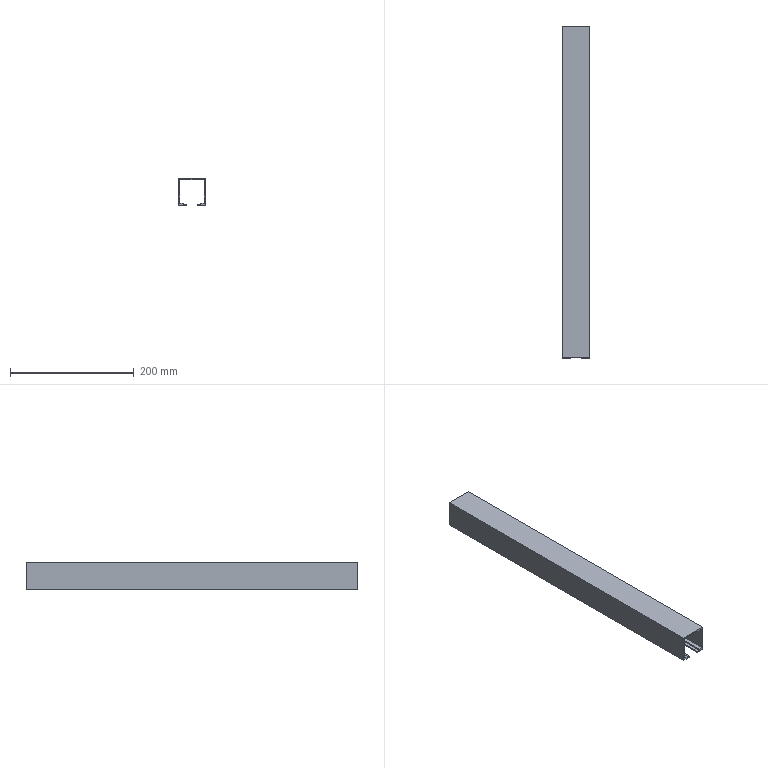Component | SolidWorks | SquareAluminumTube-2 | 1 solid | 18 faces | box 44 x 536 x 44 mm | volume 173664 mm3 | plane 18
build123d program:
from build123d import *

# Parameters (mm, degrees)
BOSS_EXTRUDE1_DEPTH = 536


with BuildPart() as part:
    # Sketch1 → Boss-Extrude1 (new body)
    with BuildSketch(Plane.XY):
        Polygon((-20, -18), (-20, 20), (20, 20), (20, -18), (14, -18), (14, -20), (9, -20), (9, -22), (22, -22), (22, 22), (-22, 22), (-22, -22), (-9, -22), (-9, -20), (-14, -20), (-14, -18), align=None)
    extrude(amount=BOSS_EXTRUDE1_DEPTH)


solid = part.part

# Placed as in the assembly
solid = solid.moved(Location((-67.793, 523.197, 1764.064), (90, 0, 0)))
STEP:
#1=CARTESIAN_POINT('',(-3.535,-0.5041,68.585));
#2=VERTEX_POINT('',#1);
#3=CARTESIAN_POINT('',(-3.535,-0.5041,70.317));
#4=VERTEX_POINT('',#3);
#5=CARTESIAN_POINT('',(-3.535,-0.5041,68.585));
#6=DIRECTION('',(0.,0.,1.));
#7=VECTOR('',#6,39.37);
#8=LINE('',#5,#7);
#9=EDGE_CURVE('',#2,#4,#8,.T.);
#10=ORIENTED_EDGE('',*,*,#9,.T.);
#11=CARTESIAN_POINT('',(-3.535,20.598,70.317));
#12=VERTEX_POINT('',#11);
#13=CARTESIAN_POINT('',(-3.535,20.598,70.317));
#14=DIRECTION('',(-0.,-1.,0.));
#15=VECTOR('',#14,39.37);
#16=LINE('',#13,#15);
#17=EDGE_CURVE('',#12,#4,#16,.T.);
#18=ORIENTED_EDGE('',*,*,#17,.F.);
#19=CARTESIAN_POINT('',(-3.535,20.598,68.585));
#20=VERTEX_POINT('',#19);
#21=CARTESIAN_POINT('',(-3.535,20.598,68.585));
#22=DIRECTION('',(0.,0.,1.));
#23=VECTOR('',#22,39.37);
#24=LINE('',#21,#23);
#25=EDGE_CURVE('',#20,#12,#24,.T.);
#26=ORIENTED_EDGE('',*,*,#25,.F.);
#27=CARTESIAN_POINT('',(-3.535,20.598,68.585));
#28=DIRECTION('',(-0.,-1.,0.));
#29=VECTOR('',#28,39.37);
#30=LINE('',#27,#29);
#31=EDGE_CURVE('',#20,#2,#30,.T.);
#32=ORIENTED_EDGE('',*,*,#31,.T.);
#33=EDGE_LOOP('',(#10,#18,#26,#32));
#34=FACE_OUTER_BOUND('',#33,.T.);
#35=CARTESIAN_POINT('',(-3.535,20.598,68.585));
#36=DIRECTION('',(1.,-0.,-0.));
#37=DIRECTION('',(0.,1.,-0.));
#38=AXIS2_PLACEMENT_3D('',#35,#36,#37);
#39=PLANE('',#38);
#40=ADVANCED_FACE('',(#34),#39,.F.);
#41=CARTESIAN_POINT('',(-1.803,-0.5041,70.317));
#42=VERTEX_POINT('',#41);
#43=CARTESIAN_POINT('',(-1.803,-0.5041,70.317));
#44=DIRECTION('',(1.,-0.,-0.));
#45=VECTOR('',#44,39.37);
#46=LINE('',#43,#45);
#47=EDGE_CURVE('',#4,#42,#46,.T.);
#48=ORIENTED_EDGE('',*,*,#47,.T.);
#49=CARTESIAN_POINT('',(-1.803,20.598,70.317));
#50=VERTEX_POINT('',#49);
#51=CARTESIAN_POINT('',(-1.803,20.598,70.317));
#52=DIRECTION('',(-0.,-1.,0.));
#53=VECTOR('',#52,39.37);
#54=LINE('',#51,#53);
#55=EDGE_CURVE('',#50,#42,#54,.T.);
#56=ORIENTED_EDGE('',*,*,#55,.F.);
#57=CARTESIAN_POINT('',(-1.803,20.598,70.317));
#58=DIRECTION('',(1.,-0.,-0.));
#59=VECTOR('',#58,39.37);
#60=LINE('',#57,#59);
#61=EDGE_CURVE('',#12,#50,#60,.T.);
#62=ORIENTED_EDGE('',*,*,#61,.F.);
#63=ORIENTED_EDGE('',*,*,#17,.T.);
#64=EDGE_LOOP('',(#48,#56,#62,#63));
#65=FACE_OUTER_BOUND('',#64,.T.);
#66=CARTESIAN_POINT('',(-1.803,20.598,70.317));
#67=DIRECTION('',(-0.,-0.,-1.));
#68=DIRECTION('',(-0.,-1.,0.));
#69=AXIS2_PLACEMENT_3D('',#66,#67,#68);
#70=PLANE('',#69);
#71=ADVANCED_FACE('',(#65),#70,.F.);
#72=CARTESIAN_POINT('',(-1.803,-0.5041,68.585));
#73=VERTEX_POINT('',#72);
#74=CARTESIAN_POINT('',(-1.803,-0.5041,68.585));
#75=DIRECTION('',(-0.,-0.,-1.));
#76=VECTOR('',#75,39.37);
#77=LINE('',#74,#76);
#78=EDGE_CURVE('',#42,#73,#77,.T.);
#79=ORIENTED_EDGE('',*,*,#78,.T.);
#80=CARTESIAN_POINT('',(-1.803,20.598,68.585));
#81=VERTEX_POINT('',#80);
#82=CARTESIAN_POINT('',(-1.803,20.598,68.585));
#83=DIRECTION('',(-0.,-1.,0.));
#84=VECTOR('',#83,39.37);
#85=LINE('',#82,#84);
#86=EDGE_CURVE('',#81,#73,#85,.T.);
#87=ORIENTED_EDGE('',*,*,#86,.F.);
#88=CARTESIAN_POINT('',(-1.803,20.598,68.585));
#89=DIRECTION('',(-0.,-0.,-1.));
#90=VECTOR('',#89,39.37);
#91=LINE('',#88,#90);
#92=EDGE_CURVE('',#50,#81,#91,.T.);
#93=ORIENTED_EDGE('',*,*,#92,.F.);
#94=ORIENTED_EDGE('',*,*,#55,.T.);
#95=EDGE_LOOP('',(#79,#87,#93,#94));
#96=FACE_OUTER_BOUND('',#95,.T.);
#97=CARTESIAN_POINT('',(-1.803,20.598,68.585));
#98=DIRECTION('',(-1.,0.,0.));
#99=DIRECTION('',(-0.,-1.,0.));
#100=AXIS2_PLACEMENT_3D('',#97,#98,#99);
#101=PLANE('',#100);
#102=ADVANCED_FACE('',(#96),#101,.F.);
#103=CARTESIAN_POINT('',(-2.315,-0.5041,68.585));
#104=VERTEX_POINT('',#103);
#105=CARTESIAN_POINT('',(-1.803,-0.5041,68.585));
#106=DIRECTION('',(-1.,0.,0.));
#107=VECTOR('',#106,39.37);
#108=LINE('',#105,#107);
#109=EDGE_CURVE('',#73,#104,#108,.T.);
#110=ORIENTED_EDGE('',*,*,#109,.T.);
#111=CARTESIAN_POINT('',(-2.315,20.598,68.585));
#112=VERTEX_POINT('',#111);
#113=CARTESIAN_POINT('',(-2.315,20.598,68.585));
#114=DIRECTION('',(-0.,-1.,0.));
#115=VECTOR('',#114,39.37);
#116=LINE('',#113,#115);
#117=EDGE_CURVE('',#112,#104,#116,.T.);
#118=ORIENTED_EDGE('',*,*,#117,.F.);
#119=CARTESIAN_POINT('',(-1.803,20.598,68.585));
#120=DIRECTION('',(-1.,0.,0.));
#121=VECTOR('',#120,39.37);
#122=LINE('',#119,#121);
#123=EDGE_CURVE('',#81,#112,#122,.T.);
#124=ORIENTED_EDGE('',*,*,#123,.F.);
#125=ORIENTED_EDGE('',*,*,#86,.T.);
#126=EDGE_LOOP('',(#110,#118,#124,#125));
#127=FACE_OUTER_BOUND('',#126,.T.);
#128=CARTESIAN_POINT('',(-1.803,20.598,68.585));
#129=DIRECTION('',(0.,0.,1.));
#130=DIRECTION('',(1.,-0.,-0.));
#131=AXIS2_PLACEMENT_3D('',#128,#129,#130);
#132=PLANE('',#131);
#133=ADVANCED_FACE('',(#127),#132,.F.);
#134=CARTESIAN_POINT('',(-2.315,-0.5041,68.664));
#135=VERTEX_POINT('',#134);
#136=CARTESIAN_POINT('',(-2.315,-0.5041,68.664));
#137=DIRECTION('',(0.,0.,1.));
#138=VECTOR('',#137,39.37);
#139=LINE('',#136,#138);
#140=EDGE_CURVE('',#104,#135,#139,.T.);
#141=ORIENTED_EDGE('',*,*,#140,.T.);
#142=CARTESIAN_POINT('',(-2.315,20.598,68.664));
#143=VERTEX_POINT('',#142);
#144=CARTESIAN_POINT('',(-2.315,20.598,68.664));
#145=DIRECTION('',(-0.,-1.,0.));
#146=VECTOR('',#145,39.37);
#147=LINE('',#144,#146);
#148=EDGE_CURVE('',#143,#135,#147,.T.);
#149=ORIENTED_EDGE('',*,*,#148,.F.);
#150=CARTESIAN_POINT('',(-2.315,20.598,68.664));
#151=DIRECTION('',(0.,0.,1.));
#152=VECTOR('',#151,39.37);
#153=LINE('',#150,#152);
#154=EDGE_CURVE('',#112,#143,#153,.T.);
#155=ORIENTED_EDGE('',*,*,#154,.F.);
#156=ORIENTED_EDGE('',*,*,#117,.T.);
#157=EDGE_LOOP('',(#141,#149,#155,#156));
#158=FACE_OUTER_BOUND('',#157,.T.);
#159=CARTESIAN_POINT('',(-2.315,20.598,68.664));
#160=DIRECTION('',(1.,-0.,-0.));
#161=DIRECTION('',(-0.,-0.,-1.));
#162=AXIS2_PLACEMENT_3D('',#159,#160,#161);
#163=PLANE('',#162);
#164=ADVANCED_FACE('',(#158),#163,.F.);
#165=CARTESIAN_POINT('',(-2.118,-0.5041,68.664));
#166=VERTEX_POINT('',#165);
#167=CARTESIAN_POINT('',(-2.118,-0.5041,68.664));
#168=DIRECTION('',(1.,-0.,-0.));
#169=VECTOR('',#168,39.37);
#170=LINE('',#167,#169);
#171=EDGE_CURVE('',#135,#166,#170,.T.);
#172=ORIENTED_EDGE('',*,*,#171,.T.);
#173=CARTESIAN_POINT('',(-2.118,20.598,68.664));
#174=VERTEX_POINT('',#173);
#175=CARTESIAN_POINT('',(-2.118,20.598,68.664));
#176=DIRECTION('',(-0.,-1.,0.));
#177=VECTOR('',#176,39.37);
#178=LINE('',#175,#177);
#179=EDGE_CURVE('',#174,#166,#178,.T.);
#180=ORIENTED_EDGE('',*,*,#179,.F.);
#181=CARTESIAN_POINT('',(-2.118,20.598,68.664));
#182=DIRECTION('',(1.,-0.,-0.));
#183=VECTOR('',#182,39.37);
#184=LINE('',#181,#183);
#185=EDGE_CURVE('',#143,#174,#184,.T.);
#186=ORIENTED_EDGE('',*,*,#185,.F.);
#187=ORIENTED_EDGE('',*,*,#148,.T.);
#188=EDGE_LOOP('',(#172,#180,#186,#187));
#189=FACE_OUTER_BOUND('',#188,.T.);
#190=CARTESIAN_POINT('',(-2.118,20.598,68.664));
#191=DIRECTION('',(-0.,-0.,-1.));
#192=DIRECTION('',(-0.,-1.,0.));
#193=AXIS2_PLACEMENT_3D('',#190,#191,#192);
#194=PLANE('',#193);
#195=ADVANCED_FACE('',(#189),#194,.F.);
#196=CARTESIAN_POINT('',(-2.118,-0.5041,68.743));
#197=VERTEX_POINT('',#196);
#198=CARTESIAN_POINT('',(-2.118,-0.5041,68.743));
#199=DIRECTION('',(-0.,0.,1.));
#200=VECTOR('',#199,39.37);
#201=LINE('',#198,#200);
#202=EDGE_CURVE('',#166,#197,#201,.T.);
#203=ORIENTED_EDGE('',*,*,#202,.T.);
#204=CARTESIAN_POINT('',(-2.118,20.598,68.743));
#205=VERTEX_POINT('',#204);
#206=CARTESIAN_POINT('',(-2.118,20.598,68.743));
#207=DIRECTION('',(-0.,-1.,0.));
#208=VECTOR('',#207,39.37);
#209=LINE('',#206,#208);
#210=EDGE_CURVE('',#205,#197,#209,.T.);
#211=ORIENTED_EDGE('',*,*,#210,.F.);
#212=CARTESIAN_POINT('',(-2.118,20.598,68.743));
#213=DIRECTION('',(-0.,0.,1.));
#214=VECTOR('',#213,39.37);
#215=LINE('',#212,#214);
#216=EDGE_CURVE('',#174,#205,#215,.T.);
#217=ORIENTED_EDGE('',*,*,#216,.F.);
#218=ORIENTED_EDGE('',*,*,#179,.T.);
#219=EDGE_LOOP('',(#203,#211,#217,#218));
#220=FACE_OUTER_BOUND('',#219,.T.);
#221=CARTESIAN_POINT('',(-2.118,20.598,68.743));
#222=DIRECTION('',(1.,-0.,0.));
#223=DIRECTION('',(0.,-0.,-1.));
#224=AXIS2_PLACEMENT_3D('',#221,#222,#223);
#225=PLANE('',#224);
#226=ADVANCED_FACE('',(#220),#225,.F.);
#227=CARTESIAN_POINT('',(-1.882,-0.5041,68.743));
#228=VERTEX_POINT('',#227);
#229=CARTESIAN_POINT('',(-1.882,-0.5041,68.743));
#230=DIRECTION('',(1.,-0.,-0.));
#231=VECTOR('',#230,39.37);
#232=LINE('',#229,#231);
#233=EDGE_CURVE('',#197,#228,#232,.T.);
#234=ORIENTED_EDGE('',*,*,#233,.T.);
#235=CARTESIAN_POINT('',(-1.882,20.598,68.743));
#236=VERTEX_POINT('',#235);
#237=CARTESIAN_POINT('',(-1.882,20.598,68.743));
#238=DIRECTION('',(-0.,-1.,0.));
#239=VECTOR('',#238,39.37);
#240=LINE('',#237,#239);
#241=EDGE_CURVE('',#236,#228,#240,.T.);
#242=ORIENTED_EDGE('',*,*,#241,.F.);
#243=CARTESIAN_POINT('',(-1.882,20.598,68.743));
#244=DIRECTION('',(1.,-0.,-0.));
#245=VECTOR('',#244,39.37);
#246=LINE('',#243,#245);
#247=EDGE_CURVE('',#205,#236,#246,.T.);
#248=ORIENTED_EDGE('',*,*,#247,.F.);
#249=ORIENTED_EDGE('',*,*,#210,.T.);
#250=EDGE_LOOP('',(#234,#242,#248,#249));
#251=FACE_OUTER_BOUND('',#250,.T.);
#252=CARTESIAN_POINT('',(-1.882,20.598,68.743));
#253=DIRECTION('',(-0.,-0.,-1.));
#254=DIRECTION('',(-1.,0.,0.));
#255=AXIS2_PLACEMENT_3D('',#252,#253,#254);
#256=PLANE('',#255);
#257=ADVANCED_FACE('',(#251),#256,.F.);
#258=CARTESIAN_POINT('',(-1.882,-0.5041,70.239));
#259=VERTEX_POINT('',#258);
#260=CARTESIAN_POINT('',(-1.882,-0.5041,68.743));
#261=DIRECTION('',(0.,0.,1.));
#262=VECTOR('',#261,39.37);
#263=LINE('',#260,#262);
#264=EDGE_CURVE('',#228,#259,#263,.T.);
#265=ORIENTED_EDGE('',*,*,#264,.T.);
#266=CARTESIAN_POINT('',(-1.882,20.598,70.239));
#267=VERTEX_POINT('',#266);
#268=CARTESIAN_POINT('',(-1.882,20.598,70.239));
#269=DIRECTION('',(-0.,-1.,0.));
#270=VECTOR('',#269,39.37);
#271=LINE('',#268,#270);
#272=EDGE_CURVE('',#267,#259,#271,.T.);
#273=ORIENTED_EDGE('',*,*,#272,.F.);
#274=CARTESIAN_POINT('',(-1.882,20.598,68.743));
#275=DIRECTION('',(0.,0.,1.));
#276=VECTOR('',#275,39.37);
#277=LINE('',#274,#276);
#278=EDGE_CURVE('',#236,#267,#277,.T.);
#279=ORIENTED_EDGE('',*,*,#278,.F.);
#280=ORIENTED_EDGE('',*,*,#241,.T.);
#281=EDGE_LOOP('',(#265,#273,#279,#280));
#282=FACE_OUTER_BOUND('',#281,.T.);
#283=CARTESIAN_POINT('',(-1.882,20.598,68.743));
#284=DIRECTION('',(1.,-0.,-0.));
#285=DIRECTION('',(-0.,-0.,-1.));
#286=AXIS2_PLACEMENT_3D('',#283,#284,#285);
#287=PLANE('',#286);
#288=ADVANCED_FACE('',(#282),#287,.F.);
#289=CARTESIAN_POINT('',(-3.456,-0.5041,70.239));
#290=VERTEX_POINT('',#289);
#291=CARTESIAN_POINT('',(-1.882,-0.5041,70.239));
#292=DIRECTION('',(-1.,0.,0.));
#293=VECTOR('',#292,39.37);
#294=LINE('',#291,#293);
#295=EDGE_CURVE('',#259,#290,#294,.T.);
#296=ORIENTED_EDGE('',*,*,#295,.T.);
#297=CARTESIAN_POINT('',(-3.456,20.598,70.239));
#298=VERTEX_POINT('',#297);
#299=CARTESIAN_POINT('',(-3.456,20.598,70.239));
#300=DIRECTION('',(-0.,-1.,0.));
#301=VECTOR('',#300,39.37);
#302=LINE('',#299,#301);
#303=EDGE_CURVE('',#298,#290,#302,.T.);
#304=ORIENTED_EDGE('',*,*,#303,.F.);
#305=CARTESIAN_POINT('',(-1.882,20.598,70.239));
#306=DIRECTION('',(-1.,0.,0.));
#307=VECTOR('',#306,39.37);
#308=LINE('',#305,#307);
#309=EDGE_CURVE('',#267,#298,#308,.T.);
#310=ORIENTED_EDGE('',*,*,#309,.F.);
#311=ORIENTED_EDGE('',*,*,#272,.T.);
#312=EDGE_LOOP('',(#296,#304,#310,#311));
#313=FACE_OUTER_BOUND('',#312,.T.);
#314=CARTESIAN_POINT('',(-1.882,20.598,70.239));
#315=DIRECTION('',(0.,0.,1.));
#316=DIRECTION('',(0.,1.,-0.));
#317=AXIS2_PLACEMENT_3D('',#314,#315,#316);
#318=PLANE('',#317);
#319=ADVANCED_FACE('',(#313),#318,.F.);
#320=CARTESIAN_POINT('',(-3.456,-0.5041,68.743));
#321=VERTEX_POINT('',#320);
#322=CARTESIAN_POINT('',(-3.456,-0.5041,68.743));
#323=DIRECTION('',(-0.,-0.,-1.));
#324=VECTOR('',#323,39.37);
#325=LINE('',#322,#324);
#326=EDGE_CURVE('',#290,#321,#325,.T.);
#327=ORIENTED_EDGE('',*,*,#326,.T.);
#328=CARTESIAN_POINT('',(-3.456,20.598,68.743));
#329=VERTEX_POINT('',#328);
#330=CARTESIAN_POINT('',(-3.456,20.598,68.743));
#331=DIRECTION('',(-0.,-1.,0.));
#332=VECTOR('',#331,39.37);
#333=LINE('',#330,#332);
#334=EDGE_CURVE('',#329,#321,#333,.T.);
#335=ORIENTED_EDGE('',*,*,#334,.F.);
#336=CARTESIAN_POINT('',(-3.456,20.598,68.743));
#337=DIRECTION('',(-0.,-0.,-1.));
#338=VECTOR('',#337,39.37);
#339=LINE('',#336,#338);
#340=EDGE_CURVE('',#298,#329,#339,.T.);
#341=ORIENTED_EDGE('',*,*,#340,.F.);
#342=ORIENTED_EDGE('',*,*,#303,.T.);
#343=EDGE_LOOP('',(#327,#335,#341,#342));
#344=FACE_OUTER_BOUND('',#343,.T.);
#345=CARTESIAN_POINT('',(-3.456,20.598,68.743));
#346=DIRECTION('',(-1.,0.,0.));
#347=DIRECTION('',(-0.,-1.,0.));
#348=AXIS2_PLACEMENT_3D('',#345,#346,#347);
#349=PLANE('',#348);
#350=ADVANCED_FACE('',(#344),#349,.F.);
#351=CARTESIAN_POINT('',(-3.22,-0.5041,68.743));
#352=VERTEX_POINT('',#351);
#353=CARTESIAN_POINT('',(-3.456,-0.5041,68.743));
#354=DIRECTION('',(1.,-0.,-0.));
#355=VECTOR('',#354,39.37);
#356=LINE('',#353,#355);
#357=EDGE_CURVE('',#321,#352,#356,.T.);
#358=ORIENTED_EDGE('',*,*,#357,.T.);
#359=CARTESIAN_POINT('',(-3.22,20.598,68.743));
#360=VERTEX_POINT('',#359);
#361=CARTESIAN_POINT('',(-3.22,20.598,68.743));
#362=DIRECTION('',(-0.,-1.,0.));
#363=VECTOR('',#362,39.37);
#364=LINE('',#361,#363);
#365=EDGE_CURVE('',#360,#352,#364,.T.);
#366=ORIENTED_EDGE('',*,*,#365,.F.);
#367=CARTESIAN_POINT('',(-3.456,20.598,68.743));
#368=DIRECTION('',(1.,-0.,-0.));
#369=VECTOR('',#368,39.37);
#370=LINE('',#367,#369);
#371=EDGE_CURVE('',#329,#360,#370,.T.);
#372=ORIENTED_EDGE('',*,*,#371,.F.);
#373=ORIENTED_EDGE('',*,*,#334,.T.);
#374=EDGE_LOOP('',(#358,#366,#372,#373));
#375=FACE_OUTER_BOUND('',#374,.T.);
#376=CARTESIAN_POINT('',(-3.456,20.598,68.743));
#377=DIRECTION('',(-0.,-0.,-1.));
#378=DIRECTION('',(-0.,-1.,0.));
#379=AXIS2_PLACEMENT_3D('',#376,#377,#378);
#380=PLANE('',#379);
#381=ADVANCED_FACE('',(#375),#380,.F.);
#382=CARTESIAN_POINT('',(-3.22,-0.5041,68.664));
#383=VERTEX_POINT('',#382);
#384=CARTESIAN_POINT('',(-3.22,-0.5041,68.743));
#385=DIRECTION('',(-0.,-0.,-1.));
#386=VECTOR('',#385,39.37);
#387=LINE('',#384,#386);
#388=EDGE_CURVE('',#352,#383,#387,.T.);
#389=ORIENTED_EDGE('',*,*,#388,.T.);
#390=CARTESIAN_POINT('',(-3.22,20.598,68.664));
#391=VERTEX_POINT('',#390);
#392=CARTESIAN_POINT('',(-3.22,20.598,68.664));
#393=DIRECTION('',(-0.,-1.,0.));
#394=VECTOR('',#393,39.37);
#395=LINE('',#392,#394);
#396=EDGE_CURVE('',#391,#383,#395,.T.);
#397=ORIENTED_EDGE('',*,*,#396,.F.);
#398=CARTESIAN_POINT('',(-3.22,20.598,68.743));
#399=DIRECTION('',(-0.,-0.,-1.));
#400=VECTOR('',#399,39.37);
#401=LINE('',#398,#400);
#402=EDGE_CURVE('',#360,#391,#401,.T.);
#403=ORIENTED_EDGE('',*,*,#402,.F.);
#404=ORIENTED_EDGE('',*,*,#365,.T.);
#405=EDGE_LOOP('',(#389,#397,#403,#404));
#406=FACE_OUTER_BOUND('',#405,.T.);
#407=CARTESIAN_POINT('',(-3.22,20.598,68.743));
#408=DIRECTION('',(-1.,0.,0.));
#409=DIRECTION('',(-0.,-1.,0.));
#410=AXIS2_PLACEMENT_3D('',#407,#408,#409);
#411=PLANE('',#410);
#412=ADVANCED_FACE('',(#406),#411,.F.);
#413=CARTESIAN_POINT('',(-3.023,-0.5041,68.664));
#414=VERTEX_POINT('',#413);
#415=CARTESIAN_POINT('',(-3.023,-0.5041,68.664));
#416=DIRECTION('',(1.,-0.,-0.));
#417=VECTOR('',#416,39.37);
#418=LINE('',#415,#417);
#419=EDGE_CURVE('',#383,#414,#418,.T.);
#420=ORIENTED_EDGE('',*,*,#419,.T.);
#421=CARTESIAN_POINT('',(-3.023,20.598,68.664));
#422=VERTEX_POINT('',#421);
#423=CARTESIAN_POINT('',(-3.023,20.598,68.664));
#424=DIRECTION('',(-0.,-1.,0.));
#425=VECTOR('',#424,39.37);
#426=LINE('',#423,#425);
#427=EDGE_CURVE('',#422,#414,#426,.T.);
#428=ORIENTED_EDGE('',*,*,#427,.F.);
#429=CARTESIAN_POINT('',(-3.023,20.598,68.664));
#430=DIRECTION('',(1.,-0.,-0.));
#431=VECTOR('',#430,39.37);
#432=LINE('',#429,#431);
#433=EDGE_CURVE('',#391,#422,#432,.T.);
#434=ORIENTED_EDGE('',*,*,#433,.F.);
#435=ORIENTED_EDGE('',*,*,#396,.T.);
#436=EDGE_LOOP('',(#420,#428,#434,#435));
#437=FACE_OUTER_BOUND('',#436,.T.);
#438=CARTESIAN_POINT('',(-3.023,20.598,68.664));
#439=DIRECTION('',(-0.,-0.,-1.));
#440=DIRECTION('',(-0.,-1.,0.));
#441=AXIS2_PLACEMENT_3D('',#438,#439,#440);
#442=PLANE('',#441);
#443=ADVANCED_FACE('',(#437),#442,.F.);
#444=CARTESIAN_POINT('',(-3.023,-0.5041,68.585));
#445=VERTEX_POINT('',#444);
#446=CARTESIAN_POINT('',(-3.023,-0.5041,68.664));
#447=DIRECTION('',(-0.,-0.,-1.));
#448=VECTOR('',#447,39.37);
#449=LINE('',#446,#448);
#450=EDGE_CURVE('',#414,#445,#449,.T.);
#451=ORIENTED_EDGE('',*,*,#450,.T.);
#452=CARTESIAN_POINT('',(-3.023,20.598,68.585));
#453=VERTEX_POINT('',#452);
#454=CARTESIAN_POINT('',(-3.023,20.598,68.585));
#455=DIRECTION('',(-0.,-1.,0.));
#456=VECTOR('',#455,39.37);
#457=LINE('',#454,#456);
#458=EDGE_CURVE('',#453,#445,#457,.T.);
#459=ORIENTED_EDGE('',*,*,#458,.F.);
#460=CARTESIAN_POINT('',(-3.023,20.598,68.664));
#461=DIRECTION('',(-0.,-0.,-1.));
#462=VECTOR('',#461,39.37);
#463=LINE('',#460,#462);
#464=EDGE_CURVE('',#422,#453,#463,.T.);
#465=ORIENTED_EDGE('',*,*,#464,.F.);
#466=ORIENTED_EDGE('',*,*,#427,.T.);
#467=EDGE_LOOP('',(#451,#459,#465,#466));
#468=FACE_OUTER_BOUND('',#467,.T.);
#469=CARTESIAN_POINT('',(-3.023,20.598,68.664));
#470=DIRECTION('',(-1.,0.,0.));
#471=DIRECTION('',(0.,0.,1.));
#472=AXIS2_PLACEMENT_3D('',#469,#470,#471);
#473=PLANE('',#472);
#474=ADVANCED_FACE('',(#468),#473,.F.);
#475=CARTESIAN_POINT('',(-3.023,-0.5041,68.585));
#476=DIRECTION('',(-1.,0.,-0.));
#477=VECTOR('',#476,39.37);
#478=LINE('',#475,#477);
#479=EDGE_CURVE('',#445,#2,#478,.T.);
#480=ORIENTED_EDGE('',*,*,#479,.T.);
#481=ORIENTED_EDGE('',*,*,#31,.F.);
#482=CARTESIAN_POINT('',(-3.023,20.598,68.585));
#483=DIRECTION('',(-1.,0.,-0.));
#484=VECTOR('',#483,39.37);
#485=LINE('',#482,#484);
#486=EDGE_CURVE('',#453,#20,#485,.T.);
#487=ORIENTED_EDGE('',*,*,#486,.F.);
#488=ORIENTED_EDGE('',*,*,#458,.T.);
#489=EDGE_LOOP('',(#480,#481,#487,#488));
#490=FACE_OUTER_BOUND('',#489,.T.);
#491=CARTESIAN_POINT('',(-3.023,20.598,68.585));
#492=DIRECTION('',(-0.,0.,1.));
#493=DIRECTION('',(1.,-0.,0.));
#494=AXIS2_PLACEMENT_3D('',#491,#492,#493);
#495=PLANE('',#494);
#496=ADVANCED_FACE('',(#490),#495,.F.);
#497=ORIENTED_EDGE('',*,*,#25,.T.);
#498=ORIENTED_EDGE('',*,*,#61,.T.);
#499=ORIENTED_EDGE('',*,*,#92,.T.);
#500=ORIENTED_EDGE('',*,*,#123,.T.);
#501=ORIENTED_EDGE('',*,*,#154,.T.);
#502=ORIENTED_EDGE('',*,*,#185,.T.);
#503=ORIENTED_EDGE('',*,*,#216,.T.);
#504=ORIENTED_EDGE('',*,*,#247,.T.);
#505=ORIENTED_EDGE('',*,*,#278,.T.);
#506=ORIENTED_EDGE('',*,*,#309,.T.);
#507=ORIENTED_EDGE('',*,*,#340,.T.);
#508=ORIENTED_EDGE('',*,*,#371,.T.);
#509=ORIENTED_EDGE('',*,*,#402,.T.);
#510=ORIENTED_EDGE('',*,*,#433,.T.);
#511=ORIENTED_EDGE('',*,*,#464,.T.);
#512=ORIENTED_EDGE('',*,*,#486,.T.);
#513=EDGE_LOOP('',(#497,#498,#499,#500,#501,#502,#503,#504,#505,#506,#507,#508,#509,#510,#511,#512));
#514=FACE_OUTER_BOUND('',#513,.T.);
#515=CARTESIAN_POINT('',(-2.669,20.598,69.451));
#516=DIRECTION('',(-0.,-1.,0.));
#517=DIRECTION('',(1.,-0.,-0.));
#518=AXIS2_PLACEMENT_3D('',#515,#516,#517);
#519=PLANE('',#518);
#520=ADVANCED_FACE('',(#514),#519,.F.);
#521=ORIENTED_EDGE('',*,*,#9,.F.);
#522=ORIENTED_EDGE('',*,*,#479,.F.);
#523=ORIENTED_EDGE('',*,*,#450,.F.);
#524=ORIENTED_EDGE('',*,*,#419,.F.);
#525=ORIENTED_EDGE('',*,*,#388,.F.);
#526=ORIENTED_EDGE('',*,*,#357,.F.);
#527=ORIENTED_EDGE('',*,*,#326,.F.);
#528=ORIENTED_EDGE('',*,*,#295,.F.);
#529=ORIENTED_EDGE('',*,*,#264,.F.);
#530=ORIENTED_EDGE('',*,*,#233,.F.);
#531=ORIENTED_EDGE('',*,*,#202,.F.);
#532=ORIENTED_EDGE('',*,*,#171,.F.);
#533=ORIENTED_EDGE('',*,*,#140,.F.);
#534=ORIENTED_EDGE('',*,*,#109,.F.);
#535=ORIENTED_EDGE('',*,*,#78,.F.);
#536=ORIENTED_EDGE('',*,*,#47,.F.);
#537=EDGE_LOOP('',(#521,#522,#523,#524,#525,#526,#527,#528,#529,#530,#531,#532,#533,#534,#535,#536));
#538=FACE_OUTER_BOUND('',#537,.T.);
#539=CARTESIAN_POINT('',(-2.669,-0.5041,69.451));
#540=DIRECTION('',(-0.,-1.,0.));
#541=DIRECTION('',(1.,-0.,-0.));
#542=AXIS2_PLACEMENT_3D('',#539,#540,#541);
#543=PLANE('',#542);
#544=ADVANCED_FACE('',(#538),#543,.T.);
#545=CLOSED_SHELL('',(#40,#71,#102,#133,#164,#195,#226,#257,#288,#319,#350,#381,#412,#443,#474,#496,#520,#544));
#546=MANIFOLD_SOLID_BREP('',#545);
#547=CARTESIAN_POINT('',(0.,0.,0.));
#548=DIRECTION('',(0.,0.,1.));
#549=DIRECTION('',(1.,0.,0.));
#550=AXIS2_PLACEMENT_3D('',#547,#548,#549);
#551=(LENGTH_UNIT()NAMED_UNIT(*)SI_UNIT($,.METRE.));
#552=LENGTH_MEASURE_WITH_UNIT(LENGTH_MEASURE(0.0254),#551);
#553=DIMENSIONAL_EXPONENTS(1.,0.,0.,0.,0.,0.,0.);
#554=(CONVERSION_BASED_UNIT('',#552)LENGTH_UNIT()NAMED_UNIT(#553));
#555=UNCERTAINTY_MEASURE_WITH_UNIT(LENGTH_MEASURE(0.00001),#554,'','');
#556=(NAMED_UNIT(*)PLANE_ANGLE_UNIT()SI_UNIT($,.RADIAN.));
#557=(NAMED_UNIT(*)SI_UNIT($,.STERADIAN.)SOLID_ANGLE_UNIT());
#558=(GEOMETRIC_REPRESENTATION_CONTEXT(3)GLOBAL_UNCERTAINTY_ASSIGNED_CONTEXT((#555))GLOBAL_UNIT_ASSIGNED_CONTEXT((#554,#556,#557))REPRESENTATION_CONTEXT('',''));
#559=ADVANCED_BREP_SHAPE_REPRESENTATION('',(#546,#550),#558);
#560=COLOUR_RGB('',0.7922,0.8196,0.9333);
#561=FILL_AREA_STYLE_COLOUR('',#560);
#562=FILL_AREA_STYLE('',(#561));
#563=SURFACE_STYLE_FILL_AREA(#562);
#564=SURFACE_SIDE_STYLE('',(#563));
#565=SURFACE_STYLE_USAGE(.BOTH.,#564);
#566=PRESENTATION_STYLE_ASSIGNMENT((#565));
#567=STYLED_ITEM('',(#566),#546);
#568=(LENGTH_UNIT()NAMED_UNIT(*)SI_UNIT($,.METRE.));
#569=LENGTH_MEASURE_WITH_UNIT(LENGTH_MEASURE(0.0254),#568);
#570=DIMENSIONAL_EXPONENTS(1.,0.,0.,0.,0.,0.,0.);
#571=(CONVERSION_BASED_UNIT('',#569)LENGTH_UNIT()NAMED_UNIT(#570));
#572=UNCERTAINTY_MEASURE_WITH_UNIT(LENGTH_MEASURE(0.00001),#571,'','');
#573=(NAMED_UNIT(*)PLANE_ANGLE_UNIT()SI_UNIT($,.RADIAN.));
#574=(NAMED_UNIT(*)SI_UNIT($,.STERADIAN.)SOLID_ANGLE_UNIT());
#575=(GEOMETRIC_REPRESENTATION_CONTEXT(3)GLOBAL_UNCERTAINTY_ASSIGNED_CONTEXT((#572))GLOBAL_UNIT_ASSIGNED_CONTEXT((#571,#573,#574))REPRESENTATION_CONTEXT('',''));
#576=MECHANICAL_DESIGN_GEOMETRIC_PRESENTATION_REPRESENTATION('',(#567),#575);
#577=PRESENTATION_LAYER_ASSIGNMENT('','',(#567));